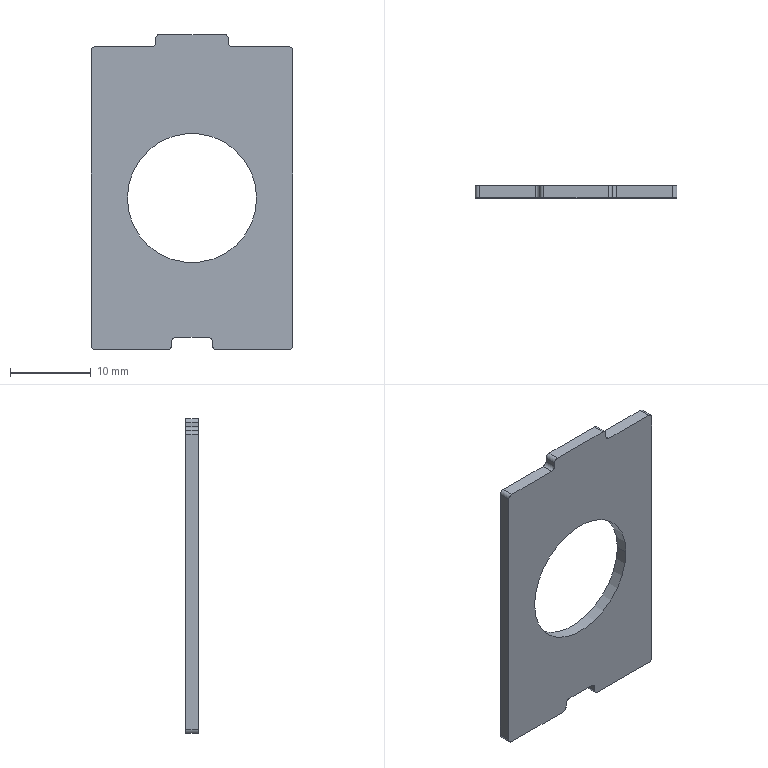Component | SolidWorks | SupportPlate-1 | 1 solid | 28 faces | box 25 x 1.5 x 39 mm | volume 1113 mm3 | cylinder 14 | plane 14 | commonest cylinder face diameters 1 x12 16 x2
build123d program:
from build123d import *

# Parameters (mm, degrees)
SKETCH1_R           = 8
BOSS_EXTRUDE2_DEPTH = 1.5
FILLET3_R           = 0.5


with BuildPart() as part:
    # Sketch1 → Boss-Extrude2 (new body)
    with BuildSketch(Plane(origin=(0, 0, 0), x_dir=(1, 0, 0), z_dir=(0, 1, 0))):
        Polygon((18.75, -4.5), (18.75, -12.5), (-18.75, -12.5), (-18.75, -2.5), (-17.25, -2.5), (-17.25, 2.5), (-18.75, 2.5), (-18.75, 12.5), (18.75, 12.5), (18.75, 4.5), (20.25, 4.5), (20.25, -4.5), align=None)
        with Locations(Location((0, 0, 0), (0, 0, 270))):
            Circle(SKETCH1_R, mode=Mode.SUBTRACT)
    extrude(amount=BOSS_EXTRUDE2_DEPTH)

    # Fillet3
    fillet3_edges = [part.edges().sort_by_distance(p)[0] for p in [
        (-18.75, 0.75, 12.5),
        (-18.75, 0.75, 2.5),
        (-17.25, 0.75, 2.5),
        (-17.25, 0.75, -2.5),
        (-18.75, 0.75, -2.5),
        (-18.75, 0.75, -12.5),
        (18.75, 0.75, -12.5),
        (18.75, 0.75, -4.5),
        (20.25, 0.75, -4.5),
        (20.25, 0.75, 4.5),
        (18.75, 0.75, 4.5),
        (18.75, 0.75, 12.5),
    ]]
    fillet(fillet3_edges, radius=FILLET3_R)


solid = part.part

# Placed as in the assembly
solid = solid.moved(Location((-50.116, 115.175, 1018.85), (0, -90, 0)))
STEP:
#1=COLOUR_RGB('',0.7922,0.8196,0.9333);
#2=FILL_AREA_STYLE_COLOUR('',#1);
#3=FILL_AREA_STYLE('',(#2));
#4=SURFACE_STYLE_FILL_AREA(#3);
#5=SURFACE_SIDE_STYLE('',(#4));
#6=SURFACE_STYLE_USAGE(.BOTH.,#5);
#7=PRESENTATION_STYLE_ASSIGNMENT((#6));
#8=CARTESIAN_POINT('',(-1.658,4.593,40.112));
#9=VERTEX_POINT('',#8);
#10=CARTESIAN_POINT('',(-2.288,4.593,40.112));
#11=VERTEX_POINT('',#10);
#12=CARTESIAN_POINT('',(-1.973,4.593,40.112));
#13=DIRECTION('',(-0.,1.,0.));
#14=DIRECTION('',(-1.,0.,0.));
#15=AXIS2_PLACEMENT_3D('',#12,#13,#14);
#16=CIRCLE('',#15,0.315);
#17=EDGE_CURVE('',#9,#11,#16,.T.);
#18=ORIENTED_EDGE('',*,*,#17,.T.);
#19=CARTESIAN_POINT('',(-2.288,4.534,40.112));
#20=VERTEX_POINT('',#19);
#21=CARTESIAN_POINT('',(-2.288,4.593,40.112));
#22=DIRECTION('',(0.,-1.,-0.));
#23=VECTOR('',#22,39.37);
#24=LINE('',#21,#23);
#25=EDGE_CURVE('',#11,#20,#24,.T.);
#26=ORIENTED_EDGE('',*,*,#25,.T.);
#27=CARTESIAN_POINT('',(-1.658,4.534,40.112));
#28=VERTEX_POINT('',#27);
#29=CARTESIAN_POINT('',(-1.973,4.534,40.112));
#30=DIRECTION('',(-0.,1.,0.));
#31=DIRECTION('',(-1.,0.,0.));
#32=AXIS2_PLACEMENT_3D('',#29,#30,#31);
#33=CIRCLE('',#32,0.315);
#34=EDGE_CURVE('',#28,#20,#33,.T.);
#35=ORIENTED_EDGE('',*,*,#34,.F.);
#36=CARTESIAN_POINT('',(-1.658,4.593,40.112));
#37=DIRECTION('',(0.,-1.,-0.));
#38=VECTOR('',#37,39.37);
#39=LINE('',#36,#38);
#40=EDGE_CURVE('',#9,#28,#39,.T.);
#41=ORIENTED_EDGE('',*,*,#40,.F.);
#42=EDGE_LOOP('',(#18,#26,#35,#41));
#43=FACE_OUTER_BOUND('',#42,.T.);
#44=CARTESIAN_POINT('',(-1.973,4.593,40.112));
#45=DIRECTION('',(0.,-1.,-0.));
#46=DIRECTION('',(1.,0.,0.));
#47=AXIS2_PLACEMENT_3D('',#44,#45,#46);
#48=CYLINDRICAL_SURFACE('',#47,0.315);
#49=ADVANCED_FACE('',(#43),#48,.F.);
#50=CARTESIAN_POINT('',(-1.481,4.593,40.831));
#51=VERTEX_POINT('',#50);
#52=CARTESIAN_POINT('',(-1.481,4.593,39.394));
#53=VERTEX_POINT('',#52);
#54=CARTESIAN_POINT('',(-1.481,4.593,39.374));
#55=DIRECTION('',(0.,0.,-1.));
#56=VECTOR('',#55,39.37);
#57=LINE('',#54,#56);
#58=EDGE_CURVE('',#51,#53,#57,.T.);
#59=ORIENTED_EDGE('',*,*,#58,.T.);
#60=CARTESIAN_POINT('',(-1.501,4.593,39.374));
#61=VERTEX_POINT('',#60);
#62=CARTESIAN_POINT('',(-1.501,4.593,39.394));
#63=DIRECTION('',(-0.,1.,0.));
#64=DIRECTION('',(1.,0.,0.));
#65=AXIS2_PLACEMENT_3D('',#62,#63,#64);
#66=CIRCLE('',#65,0.01969);
#67=EDGE_CURVE('',#53,#61,#66,.T.);
#68=ORIENTED_EDGE('',*,*,#67,.T.);
#69=CARTESIAN_POINT('',(-1.855,4.593,39.374));
#70=VERTEX_POINT('',#69);
#71=CARTESIAN_POINT('',(-1.481,4.593,39.374));
#72=DIRECTION('',(-1.,0.,-0.));
#73=VECTOR('',#72,39.37);
#74=LINE('',#71,#73);
#75=EDGE_CURVE('',#61,#70,#74,.T.);
#76=ORIENTED_EDGE('',*,*,#75,.T.);
#77=CARTESIAN_POINT('',(-1.875,4.593,39.394));
#78=VERTEX_POINT('',#77);
#79=CARTESIAN_POINT('',(-1.855,4.593,39.394));
#80=DIRECTION('',(-0.,1.,0.));
#81=DIRECTION('',(1.,0.,0.));
#82=AXIS2_PLACEMENT_3D('',#79,#80,#81);
#83=CIRCLE('',#82,0.01969);
#84=EDGE_CURVE('',#70,#78,#83,.T.);
#85=ORIENTED_EDGE('',*,*,#84,.T.);
#86=CARTESIAN_POINT('',(-1.875,4.593,39.413));
#87=VERTEX_POINT('',#86);
#88=CARTESIAN_POINT('',(-1.875,4.593,39.374));
#89=DIRECTION('',(0.,-0.,1.));
#90=VECTOR('',#89,39.37);
#91=LINE('',#88,#90);
#92=EDGE_CURVE('',#78,#87,#91,.T.);
#93=ORIENTED_EDGE('',*,*,#92,.T.);
#94=CARTESIAN_POINT('',(-1.894,4.593,39.433));
#95=VERTEX_POINT('',#94);
#96=CARTESIAN_POINT('',(-1.894,4.593,39.413));
#97=DIRECTION('',(0.,-1.,-0.));
#98=DIRECTION('',(1.,0.,0.));
#99=AXIS2_PLACEMENT_3D('',#96,#97,#98);
#100=CIRCLE('',#99,0.01969);
#101=EDGE_CURVE('',#87,#95,#100,.T.);
#102=ORIENTED_EDGE('',*,*,#101,.T.);
#103=CARTESIAN_POINT('',(-2.052,4.593,39.433));
#104=VERTEX_POINT('',#103);
#105=CARTESIAN_POINT('',(-1.875,4.593,39.433));
#106=DIRECTION('',(-1.,0.,-0.));
#107=VECTOR('',#106,39.37);
#108=LINE('',#105,#107);
#109=EDGE_CURVE('',#95,#104,#108,.T.);
#110=ORIENTED_EDGE('',*,*,#109,.T.);
#111=CARTESIAN_POINT('',(-2.072,4.593,39.413));
#112=VERTEX_POINT('',#111);
#113=CARTESIAN_POINT('',(-2.052,4.593,39.413));
#114=DIRECTION('',(0.,-1.,-0.));
#115=DIRECTION('',(1.,0.,0.));
#116=AXIS2_PLACEMENT_3D('',#113,#114,#115);
#117=CIRCLE('',#116,0.01969);
#118=EDGE_CURVE('',#104,#112,#117,.T.);
#119=ORIENTED_EDGE('',*,*,#118,.T.);
#120=CARTESIAN_POINT('',(-2.072,4.593,39.394));
#121=VERTEX_POINT('',#120);
#122=CARTESIAN_POINT('',(-2.072,4.593,39.374));
#123=DIRECTION('',(-0.,0.,-1.));
#124=VECTOR('',#123,39.37);
#125=LINE('',#122,#124);
#126=EDGE_CURVE('',#112,#121,#125,.T.);
#127=ORIENTED_EDGE('',*,*,#126,.T.);
#128=CARTESIAN_POINT('',(-2.091,4.593,39.374));
#129=VERTEX_POINT('',#128);
#130=CARTESIAN_POINT('',(-2.091,4.593,39.394));
#131=DIRECTION('',(-0.,1.,0.));
#132=DIRECTION('',(1.,0.,0.));
#133=AXIS2_PLACEMENT_3D('',#130,#131,#132);
#134=CIRCLE('',#133,0.01969);
#135=EDGE_CURVE('',#121,#129,#134,.T.);
#136=ORIENTED_EDGE('',*,*,#135,.T.);
#137=CARTESIAN_POINT('',(-2.446,4.593,39.374));
#138=VERTEX_POINT('',#137);
#139=CARTESIAN_POINT('',(-2.072,4.593,39.374));
#140=DIRECTION('',(-1.,0.,-0.));
#141=VECTOR('',#140,39.37);
#142=LINE('',#139,#141);
#143=EDGE_CURVE('',#129,#138,#142,.T.);
#144=ORIENTED_EDGE('',*,*,#143,.T.);
#145=CARTESIAN_POINT('',(-2.465,4.593,39.394));
#146=VERTEX_POINT('',#145);
#147=CARTESIAN_POINT('',(-2.446,4.593,39.394));
#148=DIRECTION('',(-0.,1.,0.));
#149=DIRECTION('',(1.,0.,0.));
#150=AXIS2_PLACEMENT_3D('',#147,#148,#149);
#151=CIRCLE('',#150,0.01969);
#152=EDGE_CURVE('',#138,#146,#151,.T.);
#153=ORIENTED_EDGE('',*,*,#152,.T.);
#154=CARTESIAN_POINT('',(-2.465,4.593,40.831));
#155=VERTEX_POINT('',#154);
#156=CARTESIAN_POINT('',(-2.465,4.593,39.374));
#157=DIRECTION('',(-0.,-0.,1.));
#158=VECTOR('',#157,39.37);
#159=LINE('',#156,#158);
#160=EDGE_CURVE('',#146,#155,#159,.T.);
#161=ORIENTED_EDGE('',*,*,#160,.T.);
#162=CARTESIAN_POINT('',(-2.446,4.593,40.85));
#163=VERTEX_POINT('',#162);
#164=CARTESIAN_POINT('',(-2.446,4.593,40.831));
#165=DIRECTION('',(-0.,1.,0.));
#166=DIRECTION('',(1.,0.,0.));
#167=AXIS2_PLACEMENT_3D('',#164,#165,#166);
#168=CIRCLE('',#167,0.01969);
#169=EDGE_CURVE('',#155,#163,#168,.T.);
#170=ORIENTED_EDGE('',*,*,#169,.T.);
#171=CARTESIAN_POINT('',(-2.17,4.593,40.85));
#172=VERTEX_POINT('',#171);
#173=CARTESIAN_POINT('',(-2.15,4.593,40.85));
#174=DIRECTION('',(1.,-0.,0.));
#175=VECTOR('',#174,39.37);
#176=LINE('',#173,#175);
#177=EDGE_CURVE('',#163,#172,#176,.T.);
#178=ORIENTED_EDGE('',*,*,#177,.T.);
#179=CARTESIAN_POINT('',(-2.15,4.593,40.87));
#180=VERTEX_POINT('',#179);
#181=CARTESIAN_POINT('',(-2.17,4.593,40.87));
#182=DIRECTION('',(0.,-1.,-0.));
#183=DIRECTION('',(1.,0.,0.));
#184=AXIS2_PLACEMENT_3D('',#181,#182,#183);
#185=CIRCLE('',#184,0.01969);
#186=EDGE_CURVE('',#172,#180,#185,.T.);
#187=ORIENTED_EDGE('',*,*,#186,.T.);
#188=CARTESIAN_POINT('',(-2.15,4.593,40.89));
#189=VERTEX_POINT('',#188);
#190=CARTESIAN_POINT('',(-2.15,4.593,40.85));
#191=DIRECTION('',(-0.,-0.,1.));
#192=VECTOR('',#191,39.37);
#193=LINE('',#190,#192);
#194=EDGE_CURVE('',#180,#189,#193,.T.);
#195=ORIENTED_EDGE('',*,*,#194,.T.);
#196=CARTESIAN_POINT('',(-2.131,4.593,40.909));
#197=VERTEX_POINT('',#196);
#198=CARTESIAN_POINT('',(-2.131,4.593,40.89));
#199=DIRECTION('',(-0.,1.,0.));
#200=DIRECTION('',(1.,0.,0.));
#201=AXIS2_PLACEMENT_3D('',#198,#199,#200);
#202=CIRCLE('',#201,0.01969);
#203=EDGE_CURVE('',#189,#197,#202,.T.);
#204=ORIENTED_EDGE('',*,*,#203,.T.);
#205=CARTESIAN_POINT('',(-1.816,4.593,40.909));
#206=VERTEX_POINT('',#205);
#207=CARTESIAN_POINT('',(-1.796,4.593,40.909));
#208=DIRECTION('',(1.,-0.,0.));
#209=VECTOR('',#208,39.37);
#210=LINE('',#207,#209);
#211=EDGE_CURVE('',#197,#206,#210,.T.);
#212=ORIENTED_EDGE('',*,*,#211,.T.);
#213=CARTESIAN_POINT('',(-1.796,4.593,40.89));
#214=VERTEX_POINT('',#213);
#215=CARTESIAN_POINT('',(-1.816,4.593,40.89));
#216=DIRECTION('',(-0.,1.,0.));
#217=DIRECTION('',(1.,0.,0.));
#218=AXIS2_PLACEMENT_3D('',#215,#216,#217);
#219=CIRCLE('',#218,0.01969);
#220=EDGE_CURVE('',#206,#214,#219,.T.);
#221=ORIENTED_EDGE('',*,*,#220,.T.);
#222=CARTESIAN_POINT('',(-1.796,4.593,40.87));
#223=VERTEX_POINT('',#222);
#224=CARTESIAN_POINT('',(-1.796,4.593,40.85));
#225=DIRECTION('',(-0.,0.,-1.));
#226=VECTOR('',#225,39.37);
#227=LINE('',#224,#226);
#228=EDGE_CURVE('',#214,#223,#227,.T.);
#229=ORIENTED_EDGE('',*,*,#228,.T.);
#230=CARTESIAN_POINT('',(-1.776,4.593,40.85));
#231=VERTEX_POINT('',#230);
#232=CARTESIAN_POINT('',(-1.776,4.593,40.87));
#233=DIRECTION('',(0.,-1.,-0.));
#234=DIRECTION('',(1.,0.,0.));
#235=AXIS2_PLACEMENT_3D('',#232,#233,#234);
#236=CIRCLE('',#235,0.01969);
#237=EDGE_CURVE('',#223,#231,#236,.T.);
#238=ORIENTED_EDGE('',*,*,#237,.T.);
#239=CARTESIAN_POINT('',(-1.501,4.593,40.85));
#240=VERTEX_POINT('',#239);
#241=CARTESIAN_POINT('',(-1.481,4.593,40.85));
#242=DIRECTION('',(1.,0.,-0.));
#243=VECTOR('',#242,39.37);
#244=LINE('',#241,#243);
#245=EDGE_CURVE('',#231,#240,#244,.T.);
#246=ORIENTED_EDGE('',*,*,#245,.T.);
#247=CARTESIAN_POINT('',(-1.501,4.593,40.831));
#248=DIRECTION('',(-0.,1.,0.));
#249=DIRECTION('',(1.,0.,0.));
#250=AXIS2_PLACEMENT_3D('',#247,#248,#249);
#251=CIRCLE('',#250,0.01969);
#252=EDGE_CURVE('',#240,#51,#251,.T.);
#253=ORIENTED_EDGE('',*,*,#252,.T.);
#254=EDGE_LOOP('',(#59,#68,#76,#85,#93,#102,#110,#119,#127,#136,#144,#153,#161,#170,#178,#187,#195,#204,#212,#221,#229,#238,#246,#253));
#255=FACE_OUTER_BOUND('',#254,.T.);
#256=ORIENTED_EDGE('',*,*,#17,.F.);
#257=CARTESIAN_POINT('',(-1.973,4.593,40.112));
#258=DIRECTION('',(-0.,1.,0.));
#259=DIRECTION('',(-1.,0.,0.));
#260=AXIS2_PLACEMENT_3D('',#257,#258,#259);
#261=CIRCLE('',#260,0.315);
#262=EDGE_CURVE('',#11,#9,#261,.T.);
#263=ORIENTED_EDGE('',*,*,#262,.F.);
#264=EDGE_LOOP('',(#256,#263));
#265=FACE_BOUND('',#264,.T.);
#266=CARTESIAN_POINT('',(-1.973,4.593,40.112));
#267=DIRECTION('',(0.,-1.,-0.));
#268=DIRECTION('',(1.,-0.,0.));
#269=AXIS2_PLACEMENT_3D('',#266,#267,#268);
#270=PLANE('',#269);
#271=ADVANCED_FACE('',(#255,#265),#270,.F.);
#272=CARTESIAN_POINT('',(-1.501,4.534,39.374));
#273=VERTEX_POINT('',#272);
#274=CARTESIAN_POINT('',(-1.855,4.534,39.374));
#275=VERTEX_POINT('',#274);
#276=CARTESIAN_POINT('',(-1.481,4.534,39.374));
#277=DIRECTION('',(-1.,0.,-0.));
#278=VECTOR('',#277,39.37);
#279=LINE('',#276,#278);
#280=EDGE_CURVE('',#273,#275,#279,.T.);
#281=ORIENTED_EDGE('',*,*,#280,.F.);
#282=CARTESIAN_POINT('',(-1.481,4.534,39.394));
#283=VERTEX_POINT('',#282);
#284=CARTESIAN_POINT('',(-1.501,4.534,39.394));
#285=DIRECTION('',(0.,-1.,-0.));
#286=DIRECTION('',(1.,0.,0.));
#287=AXIS2_PLACEMENT_3D('',#284,#285,#286);
#288=CIRCLE('',#287,0.01969);
#289=EDGE_CURVE('',#273,#283,#288,.T.);
#290=ORIENTED_EDGE('',*,*,#289,.T.);
#291=CARTESIAN_POINT('',(-1.481,4.534,40.831));
#292=VERTEX_POINT('',#291);
#293=CARTESIAN_POINT('',(-1.481,4.534,39.374));
#294=DIRECTION('',(0.,0.,-1.));
#295=VECTOR('',#294,39.37);
#296=LINE('',#293,#295);
#297=EDGE_CURVE('',#292,#283,#296,.T.);
#298=ORIENTED_EDGE('',*,*,#297,.F.);
#299=CARTESIAN_POINT('',(-1.501,4.534,40.85));
#300=VERTEX_POINT('',#299);
#301=CARTESIAN_POINT('',(-1.501,4.534,40.831));
#302=DIRECTION('',(0.,-1.,-0.));
#303=DIRECTION('',(1.,0.,0.));
#304=AXIS2_PLACEMENT_3D('',#301,#302,#303);
#305=CIRCLE('',#304,0.01969);
#306=EDGE_CURVE('',#292,#300,#305,.T.);
#307=ORIENTED_EDGE('',*,*,#306,.T.);
#308=CARTESIAN_POINT('',(-1.776,4.534,40.85));
#309=VERTEX_POINT('',#308);
#310=CARTESIAN_POINT('',(-1.481,4.534,40.85));
#311=DIRECTION('',(1.,0.,-0.));
#312=VECTOR('',#311,39.37);
#313=LINE('',#310,#312);
#314=EDGE_CURVE('',#309,#300,#313,.T.);
#315=ORIENTED_EDGE('',*,*,#314,.F.);
#316=CARTESIAN_POINT('',(-1.796,4.534,40.87));
#317=VERTEX_POINT('',#316);
#318=CARTESIAN_POINT('',(-1.776,4.534,40.87));
#319=DIRECTION('',(-0.,1.,0.));
#320=DIRECTION('',(1.,0.,0.));
#321=AXIS2_PLACEMENT_3D('',#318,#319,#320);
#322=CIRCLE('',#321,0.01969);
#323=EDGE_CURVE('',#309,#317,#322,.T.);
#324=ORIENTED_EDGE('',*,*,#323,.T.);
#325=CARTESIAN_POINT('',(-1.796,4.534,40.89));
#326=VERTEX_POINT('',#325);
#327=CARTESIAN_POINT('',(-1.796,4.534,40.85));
#328=DIRECTION('',(-0.,0.,-1.));
#329=VECTOR('',#328,39.37);
#330=LINE('',#327,#329);
#331=EDGE_CURVE('',#326,#317,#330,.T.);
#332=ORIENTED_EDGE('',*,*,#331,.F.);
#333=CARTESIAN_POINT('',(-1.816,4.534,40.909));
#334=VERTEX_POINT('',#333);
#335=CARTESIAN_POINT('',(-1.816,4.534,40.89));
#336=DIRECTION('',(0.,-1.,-0.));
#337=DIRECTION('',(1.,0.,0.));
#338=AXIS2_PLACEMENT_3D('',#335,#336,#337);
#339=CIRCLE('',#338,0.01969);
#340=EDGE_CURVE('',#326,#334,#339,.T.);
#341=ORIENTED_EDGE('',*,*,#340,.T.);
#342=CARTESIAN_POINT('',(-2.131,4.534,40.909));
#343=VERTEX_POINT('',#342);
#344=CARTESIAN_POINT('',(-1.796,4.534,40.909));
#345=DIRECTION('',(1.,-0.,0.));
#346=VECTOR('',#345,39.37);
#347=LINE('',#344,#346);
#348=EDGE_CURVE('',#343,#334,#347,.T.);
#349=ORIENTED_EDGE('',*,*,#348,.F.);
#350=CARTESIAN_POINT('',(-2.15,4.534,40.89));
#351=VERTEX_POINT('',#350);
#352=CARTESIAN_POINT('',(-2.131,4.534,40.89));
#353=DIRECTION('',(0.,-1.,-0.));
#354=DIRECTION('',(1.,0.,0.));
#355=AXIS2_PLACEMENT_3D('',#352,#353,#354);
#356=CIRCLE('',#355,0.01969);
#357=EDGE_CURVE('',#343,#351,#356,.T.);
#358=ORIENTED_EDGE('',*,*,#357,.T.);
#359=CARTESIAN_POINT('',(-2.15,4.534,40.87));
#360=VERTEX_POINT('',#359);
#361=CARTESIAN_POINT('',(-2.15,4.534,40.85));
#362=DIRECTION('',(-0.,-0.,1.));
#363=VECTOR('',#362,39.37);
#364=LINE('',#361,#363);
#365=EDGE_CURVE('',#360,#351,#364,.T.);
#366=ORIENTED_EDGE('',*,*,#365,.F.);
#367=CARTESIAN_POINT('',(-2.17,4.534,40.85));
#368=VERTEX_POINT('',#367);
#369=CARTESIAN_POINT('',(-2.17,4.534,40.87));
#370=DIRECTION('',(-0.,1.,0.));
#371=DIRECTION('',(1.,0.,0.));
#372=AXIS2_PLACEMENT_3D('',#369,#370,#371);
#373=CIRCLE('',#372,0.01969);
#374=EDGE_CURVE('',#360,#368,#373,.T.);
#375=ORIENTED_EDGE('',*,*,#374,.T.);
#376=CARTESIAN_POINT('',(-2.446,4.534,40.85));
#377=VERTEX_POINT('',#376);
#378=CARTESIAN_POINT('',(-2.15,4.534,40.85));
#379=DIRECTION('',(1.,-0.,0.));
#380=VECTOR('',#379,39.37);
#381=LINE('',#378,#380);
#382=EDGE_CURVE('',#377,#368,#381,.T.);
#383=ORIENTED_EDGE('',*,*,#382,.F.);
#384=CARTESIAN_POINT('',(-2.465,4.534,40.831));
#385=VERTEX_POINT('',#384);
#386=CARTESIAN_POINT('',(-2.446,4.534,40.831));
#387=DIRECTION('',(0.,-1.,-0.));
#388=DIRECTION('',(1.,0.,0.));
#389=AXIS2_PLACEMENT_3D('',#386,#387,#388);
#390=CIRCLE('',#389,0.01969);
#391=EDGE_CURVE('',#377,#385,#390,.T.);
#392=ORIENTED_EDGE('',*,*,#391,.T.);
#393=CARTESIAN_POINT('',(-2.465,4.534,39.394));
#394=VERTEX_POINT('',#393);
#395=CARTESIAN_POINT('',(-2.465,4.534,39.374));
#396=DIRECTION('',(-0.,-0.,1.));
#397=VECTOR('',#396,39.37);
#398=LINE('',#395,#397);
#399=EDGE_CURVE('',#394,#385,#398,.T.);
#400=ORIENTED_EDGE('',*,*,#399,.F.);
#401=CARTESIAN_POINT('',(-2.446,4.534,39.374));
#402=VERTEX_POINT('',#401);
#403=CARTESIAN_POINT('',(-2.446,4.534,39.394));
#404=DIRECTION('',(0.,-1.,-0.));
#405=DIRECTION('',(1.,0.,0.));
#406=AXIS2_PLACEMENT_3D('',#403,#404,#405);
#407=CIRCLE('',#406,0.01969);
#408=EDGE_CURVE('',#394,#402,#407,.T.);
#409=ORIENTED_EDGE('',*,*,#408,.T.);
#410=CARTESIAN_POINT('',(-2.091,4.534,39.374));
#411=VERTEX_POINT('',#410);
#412=CARTESIAN_POINT('',(-2.072,4.534,39.374));
#413=DIRECTION('',(-1.,0.,-0.));
#414=VECTOR('',#413,39.37);
#415=LINE('',#412,#414);
#416=EDGE_CURVE('',#411,#402,#415,.T.);
#417=ORIENTED_EDGE('',*,*,#416,.F.);
#418=CARTESIAN_POINT('',(-2.072,4.534,39.394));
#419=VERTEX_POINT('',#418);
#420=CARTESIAN_POINT('',(-2.091,4.534,39.394));
#421=DIRECTION('',(0.,-1.,-0.));
#422=DIRECTION('',(1.,0.,0.));
#423=AXIS2_PLACEMENT_3D('',#420,#421,#422);
#424=CIRCLE('',#423,0.01969);
#425=EDGE_CURVE('',#411,#419,#424,.T.);
#426=ORIENTED_EDGE('',*,*,#425,.T.);
#427=CARTESIAN_POINT('',(-2.072,4.534,39.413));
#428=VERTEX_POINT('',#427);
#429=CARTESIAN_POINT('',(-2.072,4.534,39.374));
#430=DIRECTION('',(-0.,0.,-1.));
#431=VECTOR('',#430,39.37);
#432=LINE('',#429,#431);
#433=EDGE_CURVE('',#428,#419,#432,.T.);
#434=ORIENTED_EDGE('',*,*,#433,.F.);
#435=CARTESIAN_POINT('',(-2.052,4.534,39.433));
#436=VERTEX_POINT('',#435);
#437=CARTESIAN_POINT('',(-2.052,4.534,39.413));
#438=DIRECTION('',(-0.,1.,0.));
#439=DIRECTION('',(1.,0.,0.));
#440=AXIS2_PLACEMENT_3D('',#437,#438,#439);
#441=CIRCLE('',#440,0.01969);
#442=EDGE_CURVE('',#428,#436,#441,.T.);
#443=ORIENTED_EDGE('',*,*,#442,.T.);
#444=CARTESIAN_POINT('',(-1.894,4.534,39.433));
#445=VERTEX_POINT('',#444);
#446=CARTESIAN_POINT('',(-1.875,4.534,39.433));
#447=DIRECTION('',(-1.,0.,-0.));
#448=VECTOR('',#447,39.37);
#449=LINE('',#446,#448);
#450=EDGE_CURVE('',#445,#436,#449,.T.);
#451=ORIENTED_EDGE('',*,*,#450,.F.);
#452=CARTESIAN_POINT('',(-1.875,4.534,39.413));
#453=VERTEX_POINT('',#452);
#454=CARTESIAN_POINT('',(-1.894,4.534,39.413));
#455=DIRECTION('',(-0.,1.,0.));
#456=DIRECTION('',(1.,0.,0.));
#457=AXIS2_PLACEMENT_3D('',#454,#455,#456);
#458=CIRCLE('',#457,0.01969);
#459=EDGE_CURVE('',#445,#453,#458,.T.);
#460=ORIENTED_EDGE('',*,*,#459,.T.);
#461=CARTESIAN_POINT('',(-1.875,4.534,39.394));
#462=VERTEX_POINT('',#461);
#463=CARTESIAN_POINT('',(-1.875,4.534,39.374));
#464=DIRECTION('',(0.,-0.,1.));
#465=VECTOR('',#464,39.37);
#466=LINE('',#463,#465);
#467=EDGE_CURVE('',#462,#453,#466,.T.);
#468=ORIENTED_EDGE('',*,*,#467,.F.);
#469=CARTESIAN_POINT('',(-1.855,4.534,39.394));
#470=DIRECTION('',(0.,-1.,-0.));
#471=DIRECTION('',(1.,0.,0.));
#472=AXIS2_PLACEMENT_3D('',#469,#470,#471);
#473=CIRCLE('',#472,0.01969);
#474=EDGE_CURVE('',#462,#275,#473,.T.);
#475=ORIENTED_EDGE('',*,*,#474,.T.);
#476=EDGE_LOOP('',(#281,#290,#298,#307,#315,#324,#332,#341,#349,#358,#366,#375,#383,#392,#400,#409,#417,#426,#434,#443,#451,#460,#468,#475));
#477=FACE_OUTER_BOUND('',#476,.T.);
#478=ORIENTED_EDGE('',*,*,#34,.T.);
#479=CARTESIAN_POINT('',(-1.973,4.534,40.112));
#480=DIRECTION('',(-0.,1.,0.));
#481=DIRECTION('',(-1.,0.,0.));
#482=AXIS2_PLACEMENT_3D('',#479,#480,#481);
#483=CIRCLE('',#482,0.315);
#484=EDGE_CURVE('',#20,#28,#483,.T.);
#485=ORIENTED_EDGE('',*,*,#484,.T.);
#486=EDGE_LOOP('',(#478,#485));
#487=FACE_BOUND('',#486,.T.);
#488=CARTESIAN_POINT('',(-1.973,4.534,40.112));
#489=DIRECTION('',(0.,-1.,-0.));
#490=DIRECTION('',(1.,-0.,0.));
#491=AXIS2_PLACEMENT_3D('',#488,#489,#490);
#492=PLANE('',#491);
#493=ADVANCED_FACE('',(#477,#487),#492,.T.);
#494=ORIENTED_EDGE('',*,*,#160,.F.);
#495=CARTESIAN_POINT('',(-2.465,4.593,39.394));
#496=DIRECTION('',(0.,-1.,-0.));
#497=VECTOR('',#496,39.37);
#498=LINE('',#495,#497);
#499=EDGE_CURVE('',#146,#394,#498,.T.);
#500=ORIENTED_EDGE('',*,*,#499,.T.);
#501=ORIENTED_EDGE('',*,*,#399,.T.);
#502=CARTESIAN_POINT('',(-2.465,4.593,40.831));
#503=DIRECTION('',(-0.,1.,0.));
#504=VECTOR('',#503,39.37);
#505=LINE('',#502,#504);
#506=EDGE_CURVE('',#385,#155,#505,.T.);
#507=ORIENTED_EDGE('',*,*,#506,.T.);
#508=EDGE_LOOP('',(#494,#500,#501,#507));
#509=FACE_OUTER_BOUND('',#508,.T.);
#510=CARTESIAN_POINT('',(-2.465,4.593,39.374));
#511=DIRECTION('',(1.,-0.,0.));
#512=DIRECTION('',(0.,0.,-1.));
#513=AXIS2_PLACEMENT_3D('',#510,#511,#512);
#514=PLANE('',#513);
#515=ADVANCED_FACE('',(#509),#514,.F.);
#516=ORIENTED_EDGE('',*,*,#177,.F.);
#517=CARTESIAN_POINT('',(-2.446,4.593,40.85));
#518=DIRECTION('',(0.,-1.,-0.));
#519=VECTOR('',#518,39.37);
#520=LINE('',#517,#519);
#521=EDGE_CURVE('',#163,#377,#520,.T.);
#522=ORIENTED_EDGE('',*,*,#521,.T.);
#523=ORIENTED_EDGE('',*,*,#382,.T.);
#524=CARTESIAN_POINT('',(-2.17,4.593,40.85));
#525=DIRECTION('',(-0.,1.,0.));
#526=VECTOR('',#525,39.37);
#527=LINE('',#524,#526);
#528=EDGE_CURVE('',#368,#172,#527,.T.);
#529=ORIENTED_EDGE('',*,*,#528,.T.);
#530=EDGE_LOOP('',(#516,#522,#523,#529));
#531=FACE_OUTER_BOUND('',#530,.T.);
#532=CARTESIAN_POINT('',(-2.15,4.593,40.85));
#533=DIRECTION('',(0.,0.,-1.));
#534=DIRECTION('',(-1.,0.,-0.));
#535=AXIS2_PLACEMENT_3D('',#532,#533,#534);
#536=PLANE('',#535);
#537=ADVANCED_FACE('',(#531),#536,.F.);
#538=ORIENTED_EDGE('',*,*,#365,.T.);
#539=CARTESIAN_POINT('',(-2.15,4.593,40.89));
#540=DIRECTION('',(-0.,1.,0.));
#541=VECTOR('',#540,39.37);
#542=LINE('',#539,#541);
#543=EDGE_CURVE('',#351,#189,#542,.T.);
#544=ORIENTED_EDGE('',*,*,#543,.T.);
#545=ORIENTED_EDGE('',*,*,#194,.F.);
#546=CARTESIAN_POINT('',(-2.15,4.534,40.87));
#547=DIRECTION('',(0.,-1.,-0.));
#548=VECTOR('',#547,39.37);
#549=LINE('',#546,#548);
#550=EDGE_CURVE('',#180,#360,#549,.T.);
#551=ORIENTED_EDGE('',*,*,#550,.T.);
#552=EDGE_LOOP('',(#538,#544,#545,#551));
#553=FACE_OUTER_BOUND('',#552,.T.);
#554=CARTESIAN_POINT('',(-2.15,4.593,40.85));
#555=DIRECTION('',(1.,-0.,0.));
#556=DIRECTION('',(0.,0.,-1.));
#557=AXIS2_PLACEMENT_3D('',#554,#555,#556);
#558=PLANE('',#557);
#559=ADVANCED_FACE('',(#553),#558,.F.);
#560=ORIENTED_EDGE('',*,*,#348,.T.);
#561=CARTESIAN_POINT('',(-1.816,4.593,40.909));
#562=DIRECTION('',(-0.,1.,0.));
#563=VECTOR('',#562,39.37);
#564=LINE('',#561,#563);
#565=EDGE_CURVE('',#334,#206,#564,.T.);
#566=ORIENTED_EDGE('',*,*,#565,.T.);
#567=ORIENTED_EDGE('',*,*,#211,.F.);
#568=CARTESIAN_POINT('',(-2.131,4.593,40.909));
#569=DIRECTION('',(0.,-1.,-0.));
#570=VECTOR('',#569,39.37);
#571=LINE('',#568,#570);
#572=EDGE_CURVE('',#197,#343,#571,.T.);
#573=ORIENTED_EDGE('',*,*,#572,.T.);
#574=EDGE_LOOP('',(#560,#566,#567,#573));
#575=FACE_OUTER_BOUND('',#574,.T.);
#576=CARTESIAN_POINT('',(-1.796,4.593,40.909));
#577=DIRECTION('',(0.,0.,-1.));
#578=DIRECTION('',(-1.,0.,-0.));
#579=AXIS2_PLACEMENT_3D('',#576,#577,#578);
#580=PLANE('',#579);
#581=ADVANCED_FACE('',(#575),#580,.F.);
#582=ORIENTED_EDGE('',*,*,#331,.T.);
#583=CARTESIAN_POINT('',(-1.796,4.593,40.87));
#584=DIRECTION('',(-0.,1.,0.));
#585=VECTOR('',#584,39.37);
#586=LINE('',#583,#585);
#587=EDGE_CURVE('',#317,#223,#586,.T.);
#588=ORIENTED_EDGE('',*,*,#587,.T.);
#589=ORIENTED_EDGE('',*,*,#228,.F.);
#590=CARTESIAN_POINT('',(-1.796,4.593,40.89));
#591=DIRECTION('',(0.,-1.,-0.));
#592=VECTOR('',#591,39.37);
#593=LINE('',#590,#592);
#594=EDGE_CURVE('',#214,#326,#593,.T.);
#595=ORIENTED_EDGE('',*,*,#594,.T.);
#596=EDGE_LOOP('',(#582,#588,#589,#595));
#597=FACE_OUTER_BOUND('',#596,.T.);
#598=CARTESIAN_POINT('',(-1.796,4.593,40.85));
#599=DIRECTION('',(-1.,-0.,0.));
#600=DIRECTION('',(0.,-0.,1.));
#601=AXIS2_PLACEMENT_3D('',#598,#599,#600);
#602=PLANE('',#601);
#603=ADVANCED_FACE('',(#597),#602,.F.);
#604=ORIENTED_EDGE('',*,*,#314,.T.);
#605=CARTESIAN_POINT('',(-1.501,4.593,40.85));
#606=DIRECTION('',(-0.,1.,0.));
#607=VECTOR('',#606,39.37);
#608=LINE('',#605,#607);
#609=EDGE_CURVE('',#300,#240,#608,.T.);
#610=ORIENTED_EDGE('',*,*,#609,.T.);
#611=ORIENTED_EDGE('',*,*,#245,.F.);
#612=CARTESIAN_POINT('',(-1.776,4.534,40.85));
#613=DIRECTION('',(0.,-1.,-0.));
#614=VECTOR('',#613,39.37);
#615=LINE('',#612,#614);
#616=EDGE_CURVE('',#231,#309,#615,.T.);
#617=ORIENTED_EDGE('',*,*,#616,.T.);
#618=EDGE_LOOP('',(#604,#610,#611,#617));
#619=FACE_OUTER_BOUND('',#618,.T.);
#620=CARTESIAN_POINT('',(-1.481,4.593,40.85));
#621=DIRECTION('',(-0.,0.,-1.));
#622=DIRECTION('',(-1.,-0.,0.));
#623=AXIS2_PLACEMENT_3D('',#620,#621,#622);
#624=PLANE('',#623);
#625=ADVANCED_FACE('',(#619),#624,.F.);
#626=ORIENTED_EDGE('',*,*,#297,.T.);
#627=CARTESIAN_POINT('',(-1.481,4.593,39.394));
#628=DIRECTION('',(-0.,1.,0.));
#629=VECTOR('',#628,39.37);
#630=LINE('',#627,#629);
#631=EDGE_CURVE('',#283,#53,#630,.T.);
#632=ORIENTED_EDGE('',*,*,#631,.T.);
#633=ORIENTED_EDGE('',*,*,#58,.F.);
#634=CARTESIAN_POINT('',(-1.481,4.593,40.831));
#635=DIRECTION('',(0.,-1.,-0.));
#636=VECTOR('',#635,39.37);
#637=LINE('',#634,#636);
#638=EDGE_CURVE('',#51,#292,#637,.T.);
#639=ORIENTED_EDGE('',*,*,#638,.T.);
#640=EDGE_LOOP('',(#626,#632,#633,#639));
#641=FACE_OUTER_BOUND('',#640,.T.);
#642=CARTESIAN_POINT('',(-1.481,4.593,39.374));
#643=DIRECTION('',(-1.,0.,-0.));
#644=DIRECTION('',(-0.,-0.,1.));
#645=AXIS2_PLACEMENT_3D('',#642,#643,#644);
#646=PLANE('',#645);
#647=ADVANCED_FACE('',(#641),#646,.F.);
#648=ORIENTED_EDGE('',*,*,#75,.F.);
#649=CARTESIAN_POINT('',(-1.501,4.593,39.374));
#650=DIRECTION('',(0.,-1.,-0.));
#651=VECTOR('',#650,39.37);
#652=LINE('',#649,#651);
#653=EDGE_CURVE('',#61,#273,#652,.T.);
#654=ORIENTED_EDGE('',*,*,#653,.T.);
#655=ORIENTED_EDGE('',*,*,#280,.T.);
#656=CARTESIAN_POINT('',(-1.855,4.593,39.374));
#657=DIRECTION('',(-0.,1.,0.));
#658=VECTOR('',#657,39.37);
#659=LINE('',#656,#658);
#660=EDGE_CURVE('',#275,#70,#659,.T.);
#661=ORIENTED_EDGE('',*,*,#660,.T.);
#662=EDGE_LOOP('',(#648,#654,#655,#661));
#663=FACE_OUTER_BOUND('',#662,.T.);
#664=CARTESIAN_POINT('',(-1.481,4.593,39.374));
#665=DIRECTION('',(-0.,-0.,1.));
#666=DIRECTION('',(1.,-0.,0.));
#667=AXIS2_PLACEMENT_3D('',#664,#665,#666);
#668=PLANE('',#667);
#669=ADVANCED_FACE('',(#663),#668,.F.);
#670=ORIENTED_EDGE('',*,*,#92,.F.);
#671=CARTESIAN_POINT('',(-1.875,4.593,39.394));
#672=DIRECTION('',(0.,-1.,-0.));
#673=VECTOR('',#672,39.37);
#674=LINE('',#671,#673);
#675=EDGE_CURVE('',#78,#462,#674,.T.);
#676=ORIENTED_EDGE('',*,*,#675,.T.);
#677=ORIENTED_EDGE('',*,*,#467,.T.);
#678=CARTESIAN_POINT('',(-1.875,4.593,39.413));
#679=DIRECTION('',(-0.,1.,0.));
#680=VECTOR('',#679,39.37);
#681=LINE('',#678,#680);
#682=EDGE_CURVE('',#453,#87,#681,.T.);
#683=ORIENTED_EDGE('',*,*,#682,.T.);
#684=EDGE_LOOP('',(#670,#676,#677,#683));
#685=FACE_OUTER_BOUND('',#684,.T.);
#686=CARTESIAN_POINT('',(-1.875,4.593,39.374));
#687=DIRECTION('',(1.,0.,-0.));
#688=DIRECTION('',(-0.,0.,-1.));
#689=AXIS2_PLACEMENT_3D('',#686,#687,#688);
#690=PLANE('',#689);
#691=ADVANCED_FACE('',(#685),#690,.F.);
#692=ORIENTED_EDGE('',*,*,#109,.F.);
#693=CARTESIAN_POINT('',(-1.894,4.534,39.433));
#694=DIRECTION('',(0.,-1.,-0.));
#695=VECTOR('',#694,39.37);
#696=LINE('',#693,#695);
#697=EDGE_CURVE('',#95,#445,#696,.T.);
#698=ORIENTED_EDGE('',*,*,#697,.T.);
#699=ORIENTED_EDGE('',*,*,#450,.T.);
#700=CARTESIAN_POINT('',(-2.052,4.593,39.433));
#701=DIRECTION('',(-0.,1.,0.));
#702=VECTOR('',#701,39.37);
#703=LINE('',#700,#702);
#704=EDGE_CURVE('',#436,#104,#703,.T.);
#705=ORIENTED_EDGE('',*,*,#704,.T.);
#706=EDGE_LOOP('',(#692,#698,#699,#705));
#707=FACE_OUTER_BOUND('',#706,.T.);
#708=CARTESIAN_POINT('',(-1.875,4.593,39.433));
#709=DIRECTION('',(-0.,-0.,1.));
#710=DIRECTION('',(1.,-0.,0.));
#711=AXIS2_PLACEMENT_3D('',#708,#709,#710);
#712=PLANE('',#711);
#713=ADVANCED_FACE('',(#707),#712,.F.);
#714=ORIENTED_EDGE('',*,*,#126,.F.);
#715=CARTESIAN_POINT('',(-2.072,4.534,39.413));
#716=DIRECTION('',(0.,-1.,-0.));
#717=VECTOR('',#716,39.37);
#718=LINE('',#715,#717);
#719=EDGE_CURVE('',#112,#428,#718,.T.);
#720=ORIENTED_EDGE('',*,*,#719,.T.);
#721=ORIENTED_EDGE('',*,*,#433,.T.);
#722=CARTESIAN_POINT('',(-2.072,4.593,39.394));
#723=DIRECTION('',(-0.,1.,0.));
#724=VECTOR('',#723,39.37);
#725=LINE('',#722,#724);
#726=EDGE_CURVE('',#419,#121,#725,.T.);
#727=ORIENTED_EDGE('',*,*,#726,.T.);
#728=EDGE_LOOP('',(#714,#720,#721,#727));
#729=FACE_OUTER_BOUND('',#728,.T.);
#730=CARTESIAN_POINT('',(-2.072,4.593,39.374));
#731=DIRECTION('',(-1.,-0.,0.));
#732=DIRECTION('',(0.,-0.,1.));
#733=AXIS2_PLACEMENT_3D('',#730,#731,#732);
#734=PLANE('',#733);
#735=ADVANCED_FACE('',(#729),#734,.F.);
#736=ORIENTED_EDGE('',*,*,#143,.F.);
#737=CARTESIAN_POINT('',(-2.091,4.593,39.374));
#738=DIRECTION('',(0.,-1.,-0.));
#739=VECTOR('',#738,39.37);
#740=LINE('',#737,#739);
#741=EDGE_CURVE('',#129,#411,#740,.T.);
#742=ORIENTED_EDGE('',*,*,#741,.T.);
#743=ORIENTED_EDGE('',*,*,#416,.T.);
#744=CARTESIAN_POINT('',(-2.446,4.593,39.374));
#745=DIRECTION('',(-0.,1.,0.));
#746=VECTOR('',#745,39.37);
#747=LINE('',#744,#746);
#748=EDGE_CURVE('',#402,#138,#747,.T.);
#749=ORIENTED_EDGE('',*,*,#748,.T.);
#750=EDGE_LOOP('',(#736,#742,#743,#749));
#751=FACE_OUTER_BOUND('',#750,.T.);
#752=CARTESIAN_POINT('',(-2.072,4.593,39.374));
#753=DIRECTION('',(-0.,-0.,1.));
#754=DIRECTION('',(1.,-0.,0.));
#755=AXIS2_PLACEMENT_3D('',#752,#753,#754);
#756=PLANE('',#755);
#757=ADVANCED_FACE('',(#751),#756,.F.);
#758=ORIENTED_EDGE('',*,*,#25,.F.);
#759=ORIENTED_EDGE('',*,*,#262,.T.);
#760=ORIENTED_EDGE('',*,*,#40,.T.);
#761=ORIENTED_EDGE('',*,*,#484,.F.);
#762=EDGE_LOOP('',(#758,#759,#760,#761));
#763=FACE_OUTER_BOUND('',#762,.T.);
#764=CARTESIAN_POINT('',(-1.973,4.593,40.112));
#765=DIRECTION('',(0.,-1.,-0.));
#766=DIRECTION('',(1.,0.,0.));
#767=AXIS2_PLACEMENT_3D('',#764,#765,#766);
#768=CYLINDRICAL_SURFACE('',#767,0.315);
#769=ADVANCED_FACE('',(#763),#768,.F.);
#770=ORIENTED_EDGE('',*,*,#67,.F.);
#771=ORIENTED_EDGE('',*,*,#631,.F.);
#772=ORIENTED_EDGE('',*,*,#289,.F.);
#773=ORIENTED_EDGE('',*,*,#653,.F.);
#774=EDGE_LOOP('',(#770,#771,#772,#773));
#775=FACE_OUTER_BOUND('',#774,.T.);
#776=CARTESIAN_POINT('',(-1.501,4.593,39.394));
#777=DIRECTION('',(0.,-1.,-0.));
#778=DIRECTION('',(1.,0.,0.));
#779=AXIS2_PLACEMENT_3D('',#776,#777,#778);
#780=CYLINDRICAL_SURFACE('',#779,0.01969);
#781=ADVANCED_FACE('',(#775),#780,.T.);
#782=ORIENTED_EDGE('',*,*,#84,.F.);
#783=ORIENTED_EDGE('',*,*,#660,.F.);
#784=ORIENTED_EDGE('',*,*,#474,.F.);
#785=ORIENTED_EDGE('',*,*,#675,.F.);
#786=EDGE_LOOP('',(#782,#783,#784,#785));
#787=FACE_OUTER_BOUND('',#786,.T.);
#788=CARTESIAN_POINT('',(-1.855,4.593,39.394));
#789=DIRECTION('',(0.,-1.,-0.));
#790=DIRECTION('',(1.,0.,0.));
#791=AXIS2_PLACEMENT_3D('',#788,#789,#790);
#792=CYLINDRICAL_SURFACE('',#791,0.01969);
#793=ADVANCED_FACE('',(#787),#792,.T.);
#794=ORIENTED_EDGE('',*,*,#101,.F.);
#795=ORIENTED_EDGE('',*,*,#682,.F.);
#796=ORIENTED_EDGE('',*,*,#459,.F.);
#797=ORIENTED_EDGE('',*,*,#697,.F.);
#798=EDGE_LOOP('',(#794,#795,#796,#797));
#799=FACE_OUTER_BOUND('',#798,.T.);
#800=CARTESIAN_POINT('',(-1.894,4.593,39.413));
#801=DIRECTION('',(-0.,1.,0.));
#802=DIRECTION('',(-1.,0.,0.));
#803=AXIS2_PLACEMENT_3D('',#800,#801,#802);
#804=CYLINDRICAL_SURFACE('',#803,0.01969);
#805=ADVANCED_FACE('',(#799),#804,.F.);
#806=ORIENTED_EDGE('',*,*,#118,.F.);
#807=ORIENTED_EDGE('',*,*,#704,.F.);
#808=ORIENTED_EDGE('',*,*,#442,.F.);
#809=ORIENTED_EDGE('',*,*,#719,.F.);
#810=EDGE_LOOP('',(#806,#807,#808,#809));
#811=FACE_OUTER_BOUND('',#810,.T.);
#812=CARTESIAN_POINT('',(-2.052,4.593,39.413));
#813=DIRECTION('',(-0.,1.,0.));
#814=DIRECTION('',(-1.,0.,0.));
#815=AXIS2_PLACEMENT_3D('',#812,#813,#814);
#816=CYLINDRICAL_SURFACE('',#815,0.01969);
#817=ADVANCED_FACE('',(#811),#816,.F.);
#818=ORIENTED_EDGE('',*,*,#135,.F.);
#819=ORIENTED_EDGE('',*,*,#726,.F.);
#820=ORIENTED_EDGE('',*,*,#425,.F.);
#821=ORIENTED_EDGE('',*,*,#741,.F.);
#822=EDGE_LOOP('',(#818,#819,#820,#821));
#823=FACE_OUTER_BOUND('',#822,.T.);
#824=CARTESIAN_POINT('',(-2.091,4.593,39.394));
#825=DIRECTION('',(0.,-1.,-0.));
#826=DIRECTION('',(1.,0.,0.));
#827=AXIS2_PLACEMENT_3D('',#824,#825,#826);
#828=CYLINDRICAL_SURFACE('',#827,0.01969);
#829=ADVANCED_FACE('',(#823),#828,.T.);
#830=ORIENTED_EDGE('',*,*,#152,.F.);
#831=ORIENTED_EDGE('',*,*,#748,.F.);
#832=ORIENTED_EDGE('',*,*,#408,.F.);
#833=ORIENTED_EDGE('',*,*,#499,.F.);
#834=EDGE_LOOP('',(#830,#831,#832,#833));
#835=FACE_OUTER_BOUND('',#834,.T.);
#836=CARTESIAN_POINT('',(-2.446,4.593,39.394));
#837=DIRECTION('',(0.,-1.,-0.));
#838=DIRECTION('',(1.,0.,0.));
#839=AXIS2_PLACEMENT_3D('',#836,#837,#838);
#840=CYLINDRICAL_SURFACE('',#839,0.01969);
#841=ADVANCED_FACE('',(#835),#840,.T.);
#842=ORIENTED_EDGE('',*,*,#169,.F.);
#843=ORIENTED_EDGE('',*,*,#506,.F.);
#844=ORIENTED_EDGE('',*,*,#391,.F.);
#845=ORIENTED_EDGE('',*,*,#521,.F.);
#846=EDGE_LOOP('',(#842,#843,#844,#845));
#847=FACE_OUTER_BOUND('',#846,.T.);
#848=CARTESIAN_POINT('',(-2.446,4.593,40.831));
#849=DIRECTION('',(0.,-1.,-0.));
#850=DIRECTION('',(1.,0.,0.));
#851=AXIS2_PLACEMENT_3D('',#848,#849,#850);
#852=CYLINDRICAL_SURFACE('',#851,0.01969);
#853=ADVANCED_FACE('',(#847),#852,.T.);
#854=ORIENTED_EDGE('',*,*,#252,.F.);
#855=ORIENTED_EDGE('',*,*,#609,.F.);
#856=ORIENTED_EDGE('',*,*,#306,.F.);
#857=ORIENTED_EDGE('',*,*,#638,.F.);
#858=EDGE_LOOP('',(#854,#855,#856,#857));
#859=FACE_OUTER_BOUND('',#858,.T.);
#860=CARTESIAN_POINT('',(-1.501,4.593,40.831));
#861=DIRECTION('',(0.,-1.,-0.));
#862=DIRECTION('',(1.,0.,0.));
#863=AXIS2_PLACEMENT_3D('',#860,#861,#862);
#864=CYLINDRICAL_SURFACE('',#863,0.01969);
#865=ADVANCED_FACE('',(#859),#864,.T.);
#866=ORIENTED_EDGE('',*,*,#237,.F.);
#867=ORIENTED_EDGE('',*,*,#587,.F.);
#868=ORIENTED_EDGE('',*,*,#323,.F.);
#869=ORIENTED_EDGE('',*,*,#616,.F.);
#870=EDGE_LOOP('',(#866,#867,#868,#869));
#871=FACE_OUTER_BOUND('',#870,.T.);
#872=CARTESIAN_POINT('',(-1.776,4.593,40.87));
#873=DIRECTION('',(-0.,1.,0.));
#874=DIRECTION('',(-1.,0.,0.));
#875=AXIS2_PLACEMENT_3D('',#872,#873,#874);
#876=CYLINDRICAL_SURFACE('',#875,0.01969);
#877=ADVANCED_FACE('',(#871),#876,.F.);
#878=ORIENTED_EDGE('',*,*,#220,.F.);
#879=ORIENTED_EDGE('',*,*,#565,.F.);
#880=ORIENTED_EDGE('',*,*,#340,.F.);
#881=ORIENTED_EDGE('',*,*,#594,.F.);
#882=EDGE_LOOP('',(#878,#879,#880,#881));
#883=FACE_OUTER_BOUND('',#882,.T.);
#884=CARTESIAN_POINT('',(-1.816,4.593,40.89));
#885=DIRECTION('',(0.,-1.,-0.));
#886=DIRECTION('',(1.,0.,0.));
#887=AXIS2_PLACEMENT_3D('',#884,#885,#886);
#888=CYLINDRICAL_SURFACE('',#887,0.01969);
#889=ADVANCED_FACE('',(#883),#888,.T.);
#890=ORIENTED_EDGE('',*,*,#203,.F.);
#891=ORIENTED_EDGE('',*,*,#543,.F.);
#892=ORIENTED_EDGE('',*,*,#357,.F.);
#893=ORIENTED_EDGE('',*,*,#572,.F.);
#894=EDGE_LOOP('',(#890,#891,#892,#893));
#895=FACE_OUTER_BOUND('',#894,.T.);
#896=CARTESIAN_POINT('',(-2.131,4.593,40.89));
#897=DIRECTION('',(0.,-1.,-0.));
#898=DIRECTION('',(1.,0.,0.));
#899=AXIS2_PLACEMENT_3D('',#896,#897,#898);
#900=CYLINDRICAL_SURFACE('',#899,0.01969);
#901=ADVANCED_FACE('',(#895),#900,.T.);
#902=ORIENTED_EDGE('',*,*,#186,.F.);
#903=ORIENTED_EDGE('',*,*,#528,.F.);
#904=ORIENTED_EDGE('',*,*,#374,.F.);
#905=ORIENTED_EDGE('',*,*,#550,.F.);
#906=EDGE_LOOP('',(#902,#903,#904,#905));
#907=FACE_OUTER_BOUND('',#906,.T.);
#908=CARTESIAN_POINT('',(-2.17,4.593,40.87));
#909=DIRECTION('',(-0.,1.,0.));
#910=DIRECTION('',(-1.,0.,0.));
#911=AXIS2_PLACEMENT_3D('',#908,#909,#910);
#912=CYLINDRICAL_SURFACE('',#911,0.01969);
#913=ADVANCED_FACE('',(#907),#912,.F.);
#914=CLOSED_SHELL('',(#49,#271,#493,#515,#537,#559,#581,#603,#625,#647,#669,#691,#713,#735,#757,#769,#781,#793,#805,#817,#829,#841,#853,#865,#877,#889,#901,#913));
#915=MANIFOLD_SOLID_BREP('',#914);
#916=STYLED_ITEM('',(#7),#915);
#917=PRESENTATION_LAYER_ASSIGNMENT('','',(#916));
#918=CARTESIAN_POINT('',(0.,0.,0.));
#919=DIRECTION('',(0.,0.,1.));
#920=DIRECTION('',(1.,0.,0.));
#921=AXIS2_PLACEMENT_3D('',#918,#919,#920);
#922=(LENGTH_UNIT()NAMED_UNIT(*)SI_UNIT($,.METRE.));
#923=LENGTH_MEASURE_WITH_UNIT(LENGTH_MEASURE(0.0254),#922);
#924=DIMENSIONAL_EXPONENTS(1.,0.,0.,0.,0.,0.,0.);
#925=(CONVERSION_BASED_UNIT('',#923)LENGTH_UNIT()NAMED_UNIT(#924));
#926=UNCERTAINTY_MEASURE_WITH_UNIT(LENGTH_MEASURE(0.00001),#925,'','');
#927=(NAMED_UNIT(*)PLANE_ANGLE_UNIT()SI_UNIT($,.RADIAN.));
#928=(NAMED_UNIT(*)SI_UNIT($,.STERADIAN.)SOLID_ANGLE_UNIT());
#929=(GEOMETRIC_REPRESENTATION_CONTEXT(3)GLOBAL_UNCERTAINTY_ASSIGNED_CONTEXT((#926))GLOBAL_UNIT_ASSIGNED_CONTEXT((#925,#927,#928))REPRESENTATION_CONTEXT('',''));
#930=ADVANCED_BREP_SHAPE_REPRESENTATION('',(#915,#921),#929);
#931=(LENGTH_UNIT()NAMED_UNIT(*)SI_UNIT($,.METRE.));
#932=LENGTH_MEASURE_WITH_UNIT(LENGTH_MEASURE(0.0254),#931);
#933=DIMENSIONAL_EXPONENTS(1.,0.,0.,0.,0.,0.,0.);
#934=(CONVERSION_BASED_UNIT('',#932)LENGTH_UNIT()NAMED_UNIT(#933));
#935=UNCERTAINTY_MEASURE_WITH_UNIT(LENGTH_MEASURE(0.00001),#934,'','');
#936=(NAMED_UNIT(*)PLANE_ANGLE_UNIT()SI_UNIT($,.RADIAN.));
#937=(NAMED_UNIT(*)SI_UNIT($,.STERADIAN.)SOLID_ANGLE_UNIT());
#938=(GEOMETRIC_REPRESENTATION_CONTEXT(3)GLOBAL_UNCERTAINTY_ASSIGNED_CONTEXT((#935))GLOBAL_UNIT_ASSIGNED_CONTEXT((#934,#936,#937))REPRESENTATION_CONTEXT('',''));
#939=MECHANICAL_DESIGN_GEOMETRIC_PRESENTATION_REPRESENTATION('',(#916),#938);